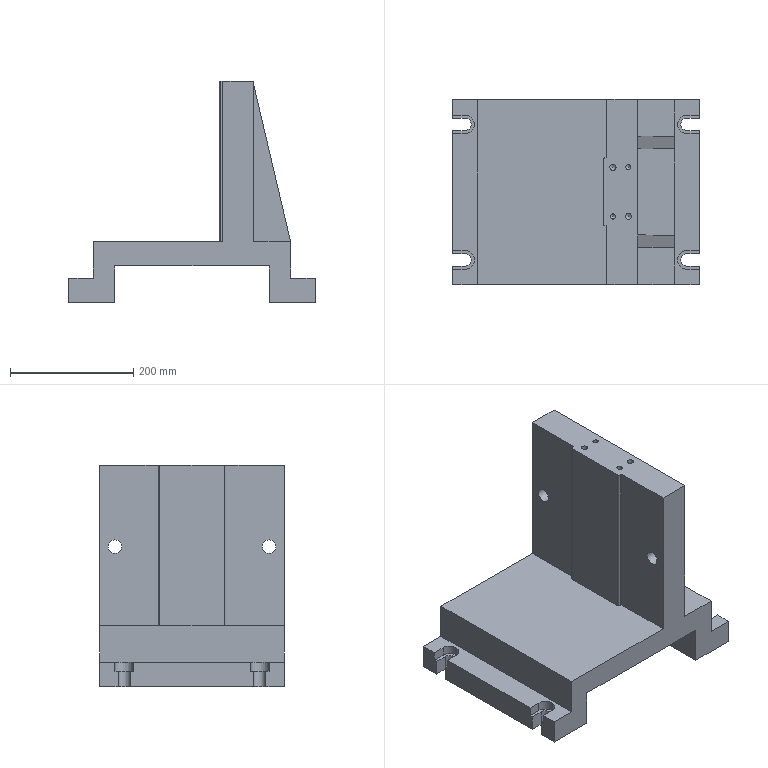Component | NX | JIG_BODY | 1 solid | 74 faces | volume 10273798 mm3 | plane 54 | cylinder 16 | cone 4 | commonest cylinder face diameters 30 x4 20 x4 6 x2 22 x2 10.006 x2 8.5 x2